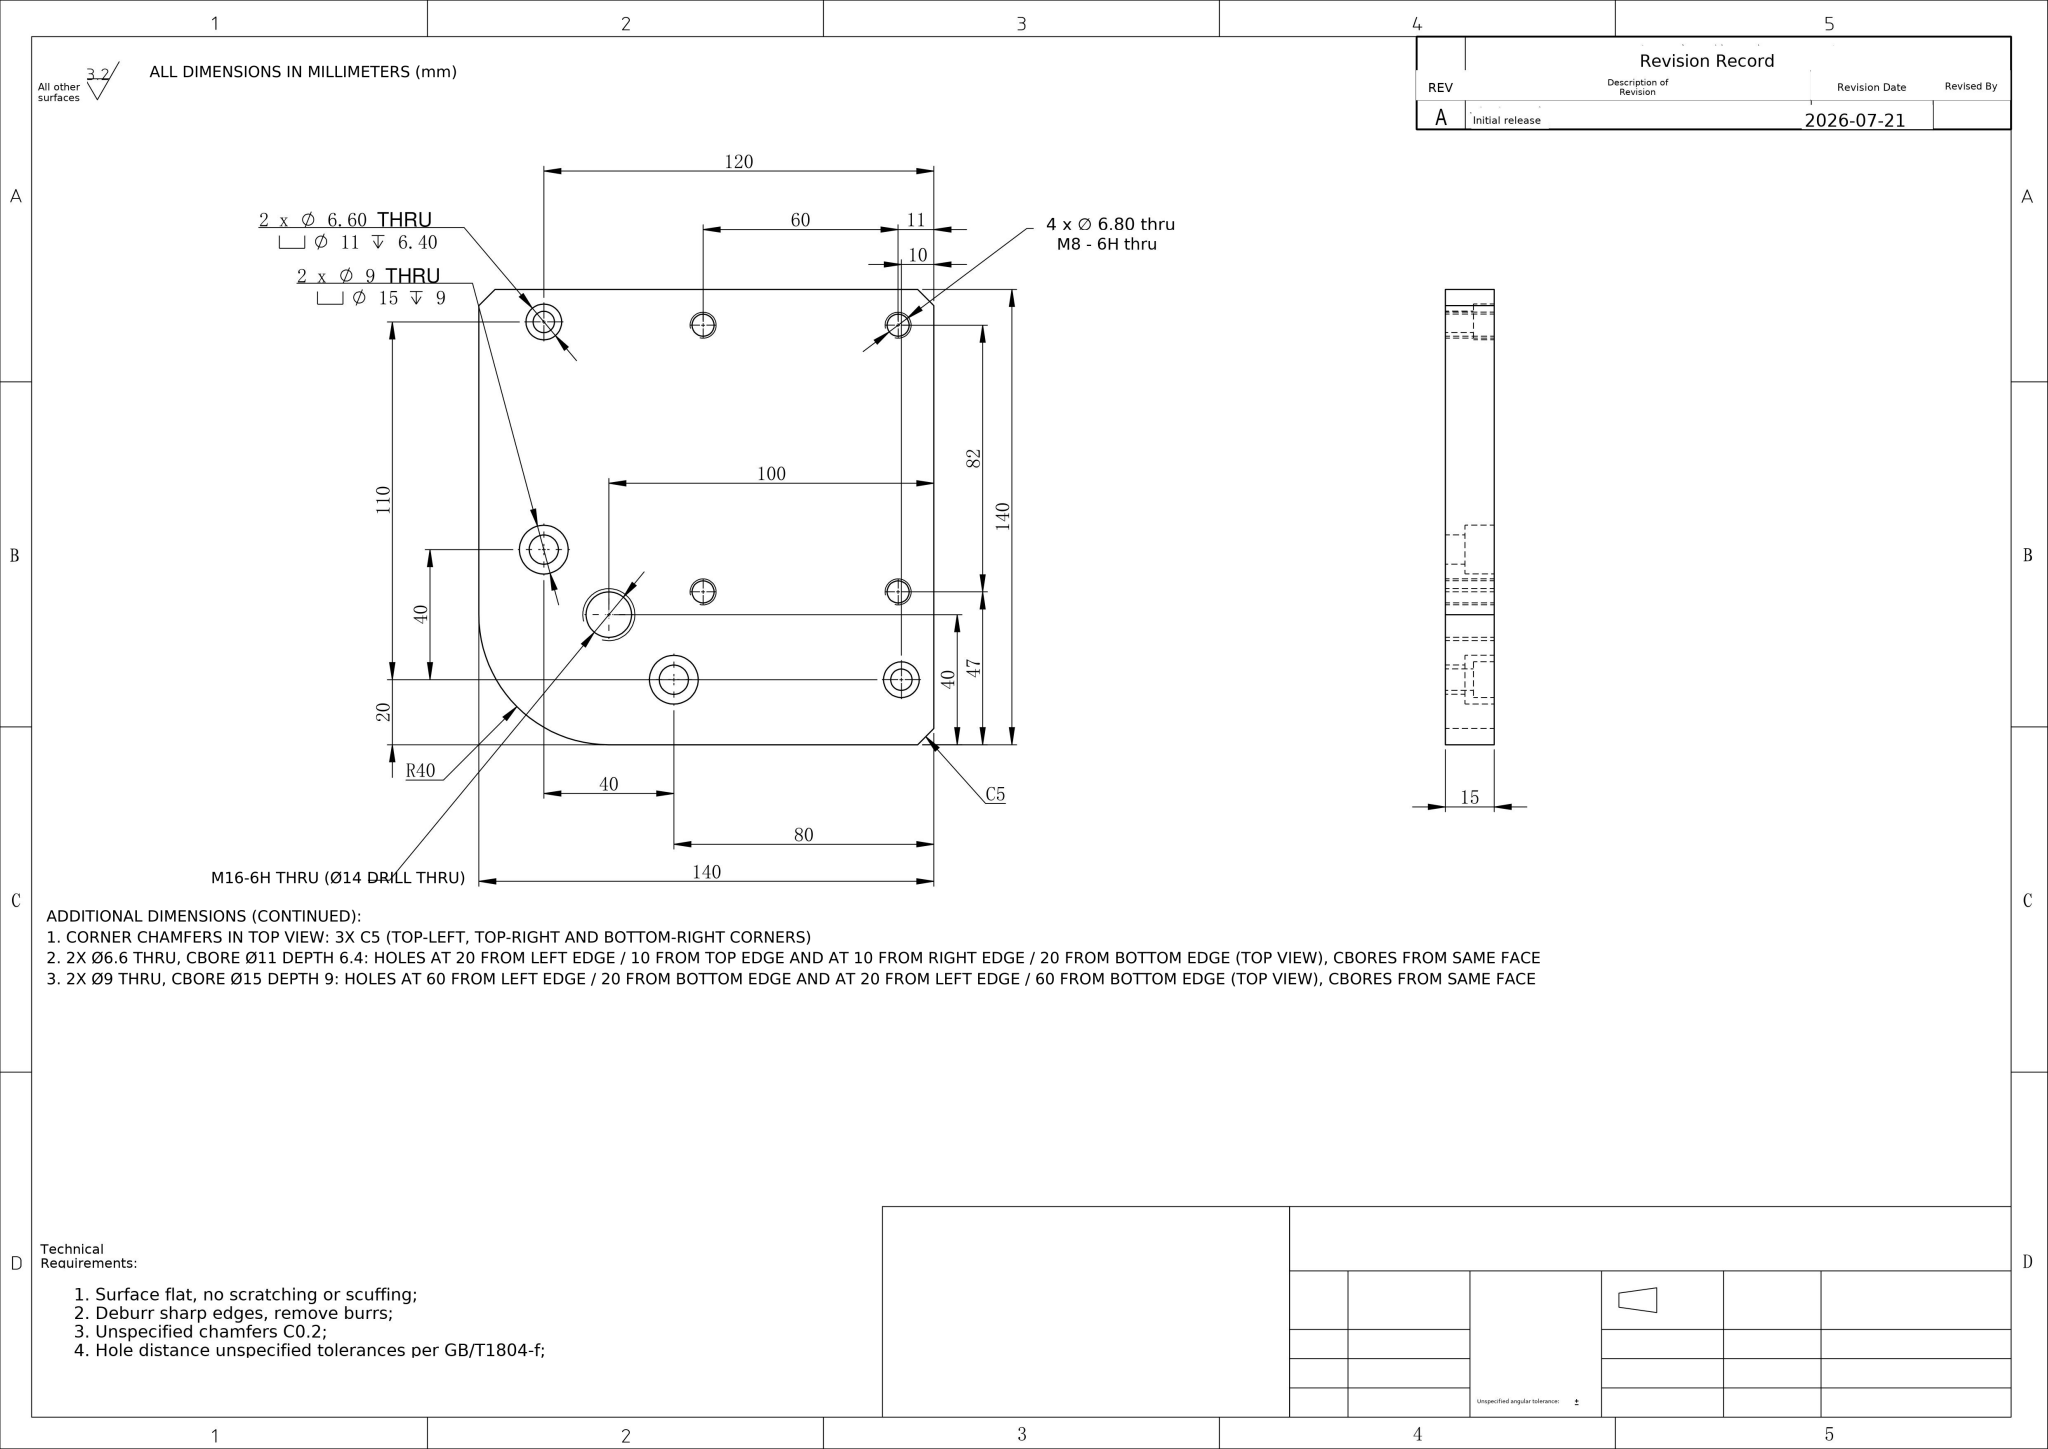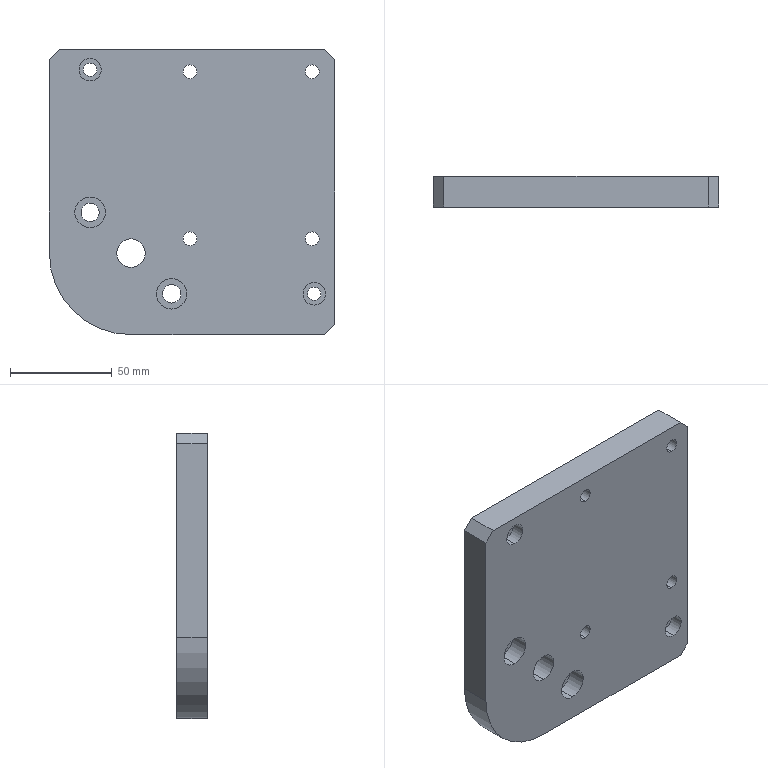Part | NX | mm | 1 solid | 40 faces | box 140 x 15 x 140 mm | volume 278050 mm3 | cylinder 27 | plane 13 | commonest cylinder face diameters 6.8 x8 15 x4 9 x4 11 x4 6.6 x4 14 x2 80 x1